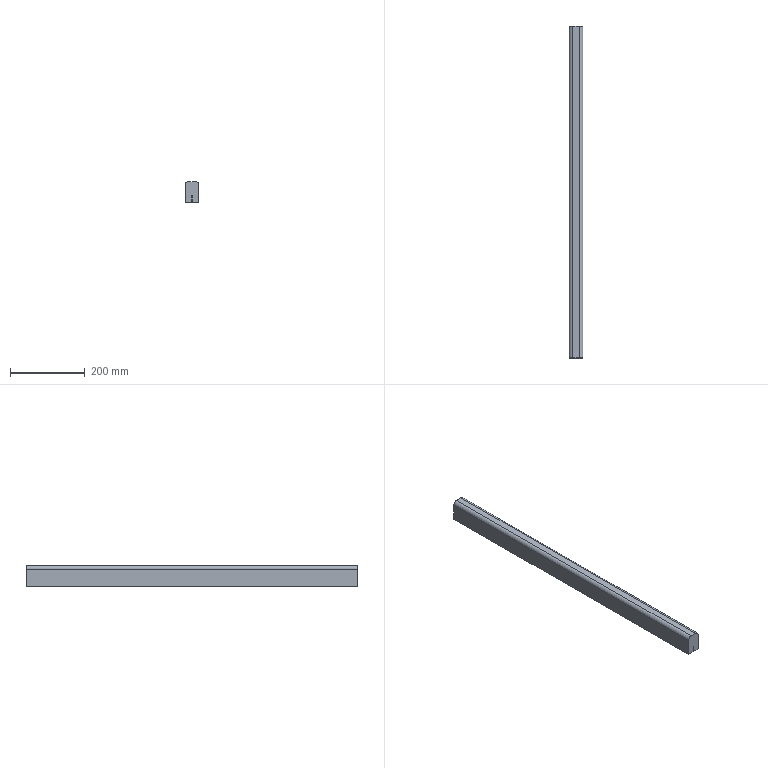Component | NX | CLOSING_ROD | 1 solid | 12 faces | box 37 x 889.3 x 56 mm | volume 1772451 mm3 | plane 10 | cylinder 2 | commonest cylinder face diameters 20 x2
STEP:
#1=CARTESIAN_POINT('',(0.,0.,0.));
#2=DIRECTION('',(0.,0.,1.));
#3=DIRECTION('',(1.,0.,0.));
#4=AXIS2_PLACEMENT_3D('',#1,#2,#3);
#5=CARTESIAN_POINT('',(344.,-444.651,-264.582));
#6=VERTEX_POINT('',#5);
#7=CARTESIAN_POINT('',(344.,444.651,-264.582));
#8=VERTEX_POINT('',#7);
#9=CARTESIAN_POINT('',(344.,-8359.443,-264.582));
#10=DIRECTION('',(0.,1.,0.));
#11=VECTOR('',#10,1.);
#12=LINE('',#9,#11);
#13=CARTESIAN_POINT('',(363.5,-8359.443,-264.582));
#14=DIRECTION('',(0.,0.,-1.));
#15=DIRECTION('',(-1.,0.,0.));
#16=AXIS2_PLACEMENT_3D('',#13,#14,#15);
#17=PLANE('',#16);
#18=CARTESIAN_POINT('',(19.5,0.));
#19=DIRECTION('',(0.,1.));
#20=VECTOR('',#19,1.);
#21=LINE('',#18,#20);
#22=(GEOMETRIC_REPRESENTATION_CONTEXT(2)PARAMETRIC_REPRESENTATION_CONTEXT()REPRESENTATION_CONTEXT('',''));
#23=DEFINITIONAL_REPRESENTATION('',(#21),#22);
#24=PCURVE('',#17,#23);
#25=CARTESIAN_POINT('',(344.,0.,-265.582));
#26=DIRECTION('',(-1.,0.,0.));
#27=DIRECTION('',(0.,0.,1.));
#28=AXIS2_PLACEMENT_3D('',#25,#26,#27);
#29=PLANE('',#28);
#30=CARTESIAN_POINT('',(1.,-8359.443));
#31=DIRECTION('',(0.,1.));
#32=VECTOR('',#31,1.);
#33=LINE('',#30,#32);
#34=(GEOMETRIC_REPRESENTATION_CONTEXT(2)PARAMETRIC_REPRESENTATION_CONTEXT()REPRESENTATION_CONTEXT('',''));
#35=DEFINITIONAL_REPRESENTATION('',(#33),#34);
#36=PCURVE('',#29,#35);
#37=SURFACE_CURVE('',#12,(#24,#36),.PCURVE_S1.);
#38=EDGE_CURVE('',#6,#8,#37,.T.);
#39=ORIENTED_EDGE('',*,*,#38,.F.);
#40=CARTESIAN_POINT('',(326.5,-444.651,-264.582));
#41=VERTEX_POINT('',#40);
#42=CARTESIAN_POINT('',(363.5,-444.651,-264.582));
#43=DIRECTION('',(1.,0.,0.));
#44=VECTOR('',#43,1.);
#45=LINE('',#42,#44);
#46=CARTESIAN_POINT('',(0.,7914.792));
#47=DIRECTION('',(-1.,0.));
#48=VECTOR('',#47,1.);
#49=LINE('',#46,#48);
#50=(GEOMETRIC_REPRESENTATION_CONTEXT(2)PARAMETRIC_REPRESENTATION_CONTEXT()REPRESENTATION_CONTEXT('',''));
#51=DEFINITIONAL_REPRESENTATION('',(#49),#50);
#52=PCURVE('',#17,#51);
#53=CARTESIAN_POINT('',(5.,-444.651,226.709));
#54=DIRECTION('',(0.,1.,0.));
#55=DIRECTION('',(0.,0.,1.));
#56=AXIS2_PLACEMENT_3D('',#53,#54,#55);
#57=PLANE('',#56);
#58=CARTESIAN_POINT('',(-491.291,358.5));
#59=DIRECTION('',(0.,1.));
#60=VECTOR('',#59,1.);
#61=LINE('',#58,#60);
#62=(GEOMETRIC_REPRESENTATION_CONTEXT(2)PARAMETRIC_REPRESENTATION_CONTEXT()REPRESENTATION_CONTEXT('',''));
#63=DEFINITIONAL_REPRESENTATION('',(#61),#62);
#64=PCURVE('',#57,#63);
#65=SURFACE_CURVE('',#45,(#52,#64),.PCURVE_S1.);
#66=EDGE_CURVE('',#41,#6,#65,.T.);
#67=ORIENTED_EDGE('',*,*,#66,.F.);
#68=CARTESIAN_POINT('',(326.5,444.651,-264.582));
#69=VERTEX_POINT('',#68);
#70=CARTESIAN_POINT('',(326.5,-8359.443,-264.582));
#71=DIRECTION('',(0.,1.,0.));
#72=VECTOR('',#71,1.);
#73=LINE('',#70,#72);
#74=CARTESIAN_POINT('',(37.,0.));
#75=DIRECTION('',(0.,1.));
#76=VECTOR('',#75,1.);
#77=LINE('',#74,#76);
#78=(GEOMETRIC_REPRESENTATION_CONTEXT(2)PARAMETRIC_REPRESENTATION_CONTEXT()REPRESENTATION_CONTEXT('',''));
#79=DEFINITIONAL_REPRESENTATION('',(#77),#78);
#80=PCURVE('',#17,#79);
#81=CARTESIAN_POINT('',(326.5,-8359.443,-249.582));
#82=DIRECTION('',(-1.,0.,0.));
#83=DIRECTION('',(0.,0.,1.));
#84=AXIS2_PLACEMENT_3D('',#81,#82,#83);
#85=PLANE('',#84);
#86=CARTESIAN_POINT('',(-15.,0.));
#87=DIRECTION('',(0.,1.));
#88=VECTOR('',#87,1.);
#89=LINE('',#86,#88);
#90=(GEOMETRIC_REPRESENTATION_CONTEXT(2)PARAMETRIC_REPRESENTATION_CONTEXT()REPRESENTATION_CONTEXT('',''));
#91=DEFINITIONAL_REPRESENTATION('',(#89),#90);
#92=PCURVE('',#85,#91);
#93=SURFACE_CURVE('',#73,(#80,#92),.PCURVE_S1.);
#94=EDGE_CURVE('',#41,#69,#93,.T.);
#95=ORIENTED_EDGE('',*,*,#94,.T.);
#96=CARTESIAN_POINT('',(363.5,444.651,-264.582));
#97=DIRECTION('',(-1.,0.,0.));
#98=VECTOR('',#97,1.);
#99=LINE('',#96,#98);
#100=CARTESIAN_POINT('',(0.,8804.095));
#101=DIRECTION('',(1.,0.));
#102=VECTOR('',#101,1.);
#103=LINE('',#100,#102);
#104=(GEOMETRIC_REPRESENTATION_CONTEXT(2)PARAMETRIC_REPRESENTATION_CONTEXT()REPRESENTATION_CONTEXT('',''));
#105=DEFINITIONAL_REPRESENTATION('',(#103),#104);
#106=PCURVE('',#17,#105);
#107=CARTESIAN_POINT('',(0.,444.651,0.));
#108=DIRECTION('',(0.,1.,0.));
#109=DIRECTION('',(0.,0.,1.));
#110=AXIS2_PLACEMENT_3D('',#107,#108,#109);
#111=PLANE('',#110);
#112=CARTESIAN_POINT('',(-264.582,363.5));
#113=DIRECTION('',(0.,-1.));
#114=VECTOR('',#113,1.);
#115=LINE('',#112,#114);
#116=(GEOMETRIC_REPRESENTATION_CONTEXT(2)PARAMETRIC_REPRESENTATION_CONTEXT()REPRESENTATION_CONTEXT('',''));
#117=DEFINITIONAL_REPRESENTATION('',(#115),#116);
#118=PCURVE('',#111,#117);
#119=SURFACE_CURVE('',#99,(#106,#118),.PCURVE_S1.);
#120=EDGE_CURVE('',#8,#69,#119,.T.);
#121=ORIENTED_EDGE('',*,*,#120,.F.);
#122=EDGE_LOOP('',(#39,#67,#95,#121));
#123=FACE_BOUND('',#122,.T.);
#124=ADVANCED_FACE('',(#123),#17,.T.);
#125=ORIENTED_EDGE('',*,*,#66,.T.);
#126=CARTESIAN_POINT('',(344.,-444.651,-246.582));
#127=VERTEX_POINT('',#126);
#128=CARTESIAN_POINT('',(344.,-444.651,226.709));
#129=DIRECTION('',(0.,0.,1.));
#130=VECTOR('',#129,1.);
#131=LINE('',#128,#130);
#132=CARTESIAN_POINT('',(0.,339.));
#133=DIRECTION('',(1.,0.));
#134=VECTOR('',#133,1.);
#135=LINE('',#132,#134);
#136=(GEOMETRIC_REPRESENTATION_CONTEXT(2)PARAMETRIC_REPRESENTATION_CONTEXT()REPRESENTATION_CONTEXT('',''));
#137=DEFINITIONAL_REPRESENTATION('',(#135),#136);
#138=PCURVE('',#57,#137);
#139=CARTESIAN_POINT('',(492.291,-444.651));
#140=DIRECTION('',(1.,0.));
#141=VECTOR('',#140,1.);
#142=LINE('',#139,#141);
#143=(GEOMETRIC_REPRESENTATION_CONTEXT(2)PARAMETRIC_REPRESENTATION_CONTEXT()REPRESENTATION_CONTEXT('',''));
#144=DEFINITIONAL_REPRESENTATION('',(#142),#143);
#145=PCURVE('',#29,#144);
#146=SURFACE_CURVE('',#131,(#138,#145),.PCURVE_S1.);
#147=EDGE_CURVE('',#6,#127,#146,.T.);
#148=ORIENTED_EDGE('',*,*,#147,.T.);
#149=CARTESIAN_POINT('',(346.,-444.651,-246.582));
#150=VERTEX_POINT('',#149);
#151=CARTESIAN_POINT('',(5.,-444.651,-246.582));
#152=DIRECTION('',(1.,0.,0.));
#153=VECTOR('',#152,1.);
#154=LINE('',#151,#153);
#155=CARTESIAN_POINT('',(-473.291,0.));
#156=DIRECTION('',(0.,1.));
#157=VECTOR('',#156,1.);
#158=LINE('',#155,#157);
#159=(GEOMETRIC_REPRESENTATION_CONTEXT(2)PARAMETRIC_REPRESENTATION_CONTEXT()REPRESENTATION_CONTEXT('',''));
#160=DEFINITIONAL_REPRESENTATION('',(#158),#159);
#161=PCURVE('',#57,#160);
#162=CARTESIAN_POINT('',(345.,0.,-246.582));
#163=DIRECTION('',(0.,0.,1.));
#164=DIRECTION('',(1.,0.,0.));
#165=AXIS2_PLACEMENT_3D('',#162,#163,#164);
#166=PLANE('',#165);
#167=CARTESIAN_POINT('',(-340.,-444.651));
#168=DIRECTION('',(1.,0.));
#169=VECTOR('',#168,1.);
#170=LINE('',#167,#169);
#171=(GEOMETRIC_REPRESENTATION_CONTEXT(2)PARAMETRIC_REPRESENTATION_CONTEXT()REPRESENTATION_CONTEXT('',''));
#172=DEFINITIONAL_REPRESENTATION('',(#170),#171);
#173=PCURVE('',#166,#172);
#174=SURFACE_CURVE('',#154,(#161,#173),.PCURVE_S1.);
#175=EDGE_CURVE('',#127,#150,#174,.T.);
#176=ORIENTED_EDGE('',*,*,#175,.T.);
#177=CARTESIAN_POINT('',(346.,-444.651,-264.582));
#178=VERTEX_POINT('',#177);
#179=CARTESIAN_POINT('',(346.,-444.651,226.709));
#180=DIRECTION('',(0.,0.,-1.));
#181=VECTOR('',#180,1.);
#182=LINE('',#179,#181);
#183=CARTESIAN_POINT('',(0.,341.));
#184=DIRECTION('',(-1.,0.));
#185=VECTOR('',#184,1.);
#186=LINE('',#183,#185);
#187=(GEOMETRIC_REPRESENTATION_CONTEXT(2)PARAMETRIC_REPRESENTATION_CONTEXT()REPRESENTATION_CONTEXT('',''));
#188=DEFINITIONAL_REPRESENTATION('',(#186),#187);
#189=PCURVE('',#57,#188);
#190=CARTESIAN_POINT('',(346.,0.,-265.582));
#191=DIRECTION('',(1.,0.,0.));
#192=DIRECTION('',(0.,0.,-1.));
#193=AXIS2_PLACEMENT_3D('',#190,#191,#192);
#194=PLANE('',#193);
#195=CARTESIAN_POINT('',(-492.291,-444.651));
#196=DIRECTION('',(1.,0.));
#197=VECTOR('',#196,1.);
#198=LINE('',#195,#197);
#199=(GEOMETRIC_REPRESENTATION_CONTEXT(2)PARAMETRIC_REPRESENTATION_CONTEXT()REPRESENTATION_CONTEXT('',''));
#200=DEFINITIONAL_REPRESENTATION('',(#198),#199);
#201=PCURVE('',#194,#200);
#202=SURFACE_CURVE('',#182,(#189,#201),.PCURVE_S1.);
#203=EDGE_CURVE('',#150,#178,#202,.T.);
#204=ORIENTED_EDGE('',*,*,#203,.T.);
#205=CARTESIAN_POINT('',(363.5,-444.651,-264.582));
#206=VERTEX_POINT('',#205);
#207=CARTESIAN_POINT('',(363.5,-444.651,-264.582));
#208=DIRECTION('',(1.,0.,0.));
#209=VECTOR('',#208,1.);
#210=LINE('',#207,#209);
#211=CARTESIAN_POINT('',(-491.291,358.5));
#212=DIRECTION('',(0.,1.));
#213=VECTOR('',#212,1.);
#214=LINE('',#211,#213);
#215=(GEOMETRIC_REPRESENTATION_CONTEXT(2)PARAMETRIC_REPRESENTATION_CONTEXT()REPRESENTATION_CONTEXT('',''));
#216=DEFINITIONAL_REPRESENTATION('',(#214),#215);
#217=PCURVE('',#57,#216);
#218=CARTESIAN_POINT('',(363.5,-8359.443,-264.582));
#219=DIRECTION('',(0.,0.,-1.));
#220=DIRECTION('',(-1.,0.,0.));
#221=AXIS2_PLACEMENT_3D('',#218,#219,#220);
#222=PLANE('',#221);
#223=CARTESIAN_POINT('',(0.,7914.792));
#224=DIRECTION('',(-1.,0.));
#225=VECTOR('',#224,1.);
#226=LINE('',#223,#225);
#227=(GEOMETRIC_REPRESENTATION_CONTEXT(2)PARAMETRIC_REPRESENTATION_CONTEXT()REPRESENTATION_CONTEXT('',''));
#228=DEFINITIONAL_REPRESENTATION('',(#226),#227);
#229=PCURVE('',#222,#228);
#230=SURFACE_CURVE('',#210,(#217,#229),.PCURVE_S1.);
#231=EDGE_CURVE('',#178,#206,#230,.T.);
#232=ORIENTED_EDGE('',*,*,#231,.T.);
#233=CARTESIAN_POINT('',(363.5,-444.651,-218.582));
#234=VERTEX_POINT('',#233);
#235=CARTESIAN_POINT('',(363.5,-444.651,-208.582));
#236=DIRECTION('',(0.,0.,1.));
#237=VECTOR('',#236,1.);
#238=LINE('',#235,#237);
#239=CARTESIAN_POINT('',(-435.291,358.5));
#240=DIRECTION('',(1.,0.));
#241=VECTOR('',#240,1.);
#242=LINE('',#239,#241);
#243=(GEOMETRIC_REPRESENTATION_CONTEXT(2)PARAMETRIC_REPRESENTATION_CONTEXT()REPRESENTATION_CONTEXT('',''));
#244=DEFINITIONAL_REPRESENTATION('',(#242),#243);
#245=PCURVE('',#57,#244);
#246=CARTESIAN_POINT('',(363.5,-8359.443,-208.582));
#247=DIRECTION('',(1.,0.,0.));
#248=DIRECTION('',(0.,0.,-1.));
#249=AXIS2_PLACEMENT_3D('',#246,#247,#248);
#250=PLANE('',#249);
#251=CARTESIAN_POINT('',(0.,7914.792));
#252=DIRECTION('',(-1.,0.));
#253=VECTOR('',#252,1.);
#254=LINE('',#251,#253);
#255=(GEOMETRIC_REPRESENTATION_CONTEXT(2)PARAMETRIC_REPRESENTATION_CONTEXT()REPRESENTATION_CONTEXT('',''));
#256=DEFINITIONAL_REPRESENTATION('',(#254),#255);
#257=PCURVE('',#250,#256);
#258=SURFACE_CURVE('',#238,(#245,#257),.PCURVE_S1.);
#259=EDGE_CURVE('',#206,#234,#258,.T.);
#260=ORIENTED_EDGE('',*,*,#259,.T.);
#261=CARTESIAN_POINT('',(353.5,-444.651,-208.582));
#262=VERTEX_POINT('',#261);
#263=CARTESIAN_POINT('',(353.5,-444.651,-218.582));
#264=DIRECTION('',(0.,-1.,0.));
#265=DIRECTION('',(0.,0.,1.));
#266=AXIS2_PLACEMENT_3D('',#263,#264,#265);
#267=CIRCLE('',#266,10.);
#268=CARTESIAN_POINT('',(-435.291,348.5));
#269=CARTESIAN_POINT('',(-435.291,331.179));
#270=CARTESIAN_POINT('',(-450.291,339.84));
#271=CARTESIAN_POINT('',(-465.291,348.5));
#272=CARTESIAN_POINT('',(-450.291,357.16));
#273=CARTESIAN_POINT('',(-435.291,365.821));
#274=CARTESIAN_POINT('',(-435.291,348.5));
#275=(BOUNDED_CURVE()B_SPLINE_CURVE(2,(#268,#269,#270,#271,#272,#273,#274),.UNSPECIFIED.,.T.,.F.)B_SPLINE_CURVE_WITH_KNOTS((1,2,2,2,2,1),(-2.094,0.,2.094,4.189,6.283,8.378),.UNSPECIFIED.)CURVE()GEOMETRIC_REPRESENTATION_ITEM()RATIONAL_B_SPLINE_CURVE((1.,0.5,1.,0.5,1.,0.5,1.))REPRESENTATION_ITEM(''));
#276=(GEOMETRIC_REPRESENTATION_CONTEXT(2)PARAMETRIC_REPRESENTATION_CONTEXT()REPRESENTATION_CONTEXT('',''));
#277=DEFINITIONAL_REPRESENTATION('',(#275),#276);
#278=PCURVE('',#57,#277);
#279=CARTESIAN_POINT('',(353.5,-8359.443,-218.582));
#280=DIRECTION('',(0.,1.,0.));
#281=DIRECTION('',(0.,0.,1.));
#282=AXIS2_PLACEMENT_3D('',#279,#280,#281);
#283=CYLINDRICAL_SURFACE('',#282,10.);
#284=CARTESIAN_POINT('',(6.283,7914.792));
#285=DIRECTION('',(-1.,0.));
#286=VECTOR('',#285,1.);
#287=LINE('',#284,#286);
#288=(GEOMETRIC_REPRESENTATION_CONTEXT(2)PARAMETRIC_REPRESENTATION_CONTEXT()REPRESENTATION_CONTEXT('',''));
#289=DEFINITIONAL_REPRESENTATION('',(#287),#288);
#290=PCURVE('',#283,#289);
#291=SURFACE_CURVE('',#267,(#278,#290),.PCURVE_S1.);
#292=EDGE_CURVE('',#234,#262,#291,.T.);
#293=ORIENTED_EDGE('',*,*,#292,.T.);
#294=CARTESIAN_POINT('',(336.5,-444.651,-208.582));
#295=VERTEX_POINT('',#294);
#296=CARTESIAN_POINT('',(326.5,-444.651,-208.582));
#297=DIRECTION('',(-1.,0.,0.));
#298=VECTOR('',#297,1.);
#299=LINE('',#296,#298);
#300=CARTESIAN_POINT('',(-435.291,321.5));
#301=DIRECTION('',(0.,-1.));
#302=VECTOR('',#301,1.);
#303=LINE('',#300,#302);
#304=(GEOMETRIC_REPRESENTATION_CONTEXT(2)PARAMETRIC_REPRESENTATION_CONTEXT()REPRESENTATION_CONTEXT('',''));
#305=DEFINITIONAL_REPRESENTATION('',(#303),#304);
#306=PCURVE('',#57,#305);
#307=CARTESIAN_POINT('',(326.5,-8359.443,-208.582));
#308=DIRECTION('',(0.,0.,1.));
#309=DIRECTION('',(1.,0.,0.));
#310=AXIS2_PLACEMENT_3D('',#307,#308,#309);
#311=PLANE('',#310);
#312=CARTESIAN_POINT('',(0.,7914.792));
#313=DIRECTION('',(-1.,0.));
#314=VECTOR('',#313,1.);
#315=LINE('',#312,#314);
#316=(GEOMETRIC_REPRESENTATION_CONTEXT(2)PARAMETRIC_REPRESENTATION_CONTEXT()REPRESENTATION_CONTEXT('',''));
#317=DEFINITIONAL_REPRESENTATION('',(#315),#316);
#318=PCURVE('',#311,#317);
#319=SURFACE_CURVE('',#299,(#306,#318),.PCURVE_S1.);
#320=EDGE_CURVE('',#262,#295,#319,.T.);
#321=ORIENTED_EDGE('',*,*,#320,.T.);
#322=CARTESIAN_POINT('',(326.5,-444.651,-218.582));
#323=VERTEX_POINT('',#322);
#324=CARTESIAN_POINT('',(336.5,-444.651,-218.582));
#325=DIRECTION('',(0.,-1.,0.));
#326=DIRECTION('',(0.,0.,1.));
#327=AXIS2_PLACEMENT_3D('',#324,#325,#326);
#328=CIRCLE('',#327,10.);
#329=CARTESIAN_POINT('',(-435.291,331.5));
#330=CARTESIAN_POINT('',(-435.291,314.179));
#331=CARTESIAN_POINT('',(-450.291,322.84));
#332=CARTESIAN_POINT('',(-465.291,331.5));
#333=CARTESIAN_POINT('',(-450.291,340.16));
#334=CARTESIAN_POINT('',(-435.291,348.821));
#335=CARTESIAN_POINT('',(-435.291,331.5));
#336=(BOUNDED_CURVE()B_SPLINE_CURVE(2,(#329,#330,#331,#332,#333,#334,#335),.UNSPECIFIED.,.T.,.F.)B_SPLINE_CURVE_WITH_KNOTS((1,2,2,2,2,1),(-2.094,0.,2.094,4.189,6.283,8.378),.UNSPECIFIED.)CURVE()GEOMETRIC_REPRESENTATION_ITEM()RATIONAL_B_SPLINE_CURVE((1.,0.5,1.,0.5,1.,0.5,1.))REPRESENTATION_ITEM(''));
#337=(GEOMETRIC_REPRESENTATION_CONTEXT(2)PARAMETRIC_REPRESENTATION_CONTEXT()REPRESENTATION_CONTEXT('',''));
#338=DEFINITIONAL_REPRESENTATION('',(#336),#337);
#339=PCURVE('',#57,#338);
#340=CARTESIAN_POINT('',(336.5,-8359.443,-218.582));
#341=DIRECTION('',(0.,1.,0.));
#342=DIRECTION('',(0.,0.,1.));
#343=AXIS2_PLACEMENT_3D('',#340,#341,#342);
#344=CYLINDRICAL_SURFACE('',#343,10.);
#345=CARTESIAN_POINT('',(6.283,7914.792));
#346=DIRECTION('',(-1.,0.));
#347=VECTOR('',#346,1.);
#348=LINE('',#345,#347);
#349=(GEOMETRIC_REPRESENTATION_CONTEXT(2)PARAMETRIC_REPRESENTATION_CONTEXT()REPRESENTATION_CONTEXT('',''));
#350=DEFINITIONAL_REPRESENTATION('',(#348),#349);
#351=PCURVE('',#344,#350);
#352=SURFACE_CURVE('',#328,(#339,#351),.PCURVE_S1.);
#353=EDGE_CURVE('',#295,#323,#352,.T.);
#354=ORIENTED_EDGE('',*,*,#353,.T.);
#355=CARTESIAN_POINT('',(326.5,-444.651,-249.582));
#356=DIRECTION('',(0.,0.,-1.));
#357=VECTOR('',#356,1.);
#358=LINE('',#355,#357);
#359=CARTESIAN_POINT('',(-476.291,321.5));
#360=DIRECTION('',(-1.,0.));
#361=VECTOR('',#360,1.);
#362=LINE('',#359,#361);
#363=(GEOMETRIC_REPRESENTATION_CONTEXT(2)PARAMETRIC_REPRESENTATION_CONTEXT()REPRESENTATION_CONTEXT('',''));
#364=DEFINITIONAL_REPRESENTATION('',(#362),#363);
#365=PCURVE('',#57,#364);
#366=CARTESIAN_POINT('',(0.,7914.792));
#367=DIRECTION('',(-1.,0.));
#368=VECTOR('',#367,1.);
#369=LINE('',#366,#368);
#370=(GEOMETRIC_REPRESENTATION_CONTEXT(2)PARAMETRIC_REPRESENTATION_CONTEXT()REPRESENTATION_CONTEXT('',''));
#371=DEFINITIONAL_REPRESENTATION('',(#369),#370);
#372=PCURVE('',#85,#371);
#373=SURFACE_CURVE('',#358,(#365,#372),.PCURVE_S1.);
#374=EDGE_CURVE('',#323,#41,#373,.T.);
#375=ORIENTED_EDGE('',*,*,#374,.T.);
#376=EDGE_LOOP('',(#125,#148,#176,#204,#232,#260,#293,#321,#354,#375));
#377=FACE_BOUND('',#376,.T.);
#378=ADVANCED_FACE('',(#377),#57,.F.);
#379=CARTESIAN_POINT('',(336.5,444.651,-208.582));
#380=VERTEX_POINT('',#379);
#381=CARTESIAN_POINT('',(353.5,444.651,-208.582));
#382=VERTEX_POINT('',#381);
#383=CARTESIAN_POINT('',(326.5,444.651,-208.582));
#384=DIRECTION('',(1.,0.,0.));
#385=VECTOR('',#384,1.);
#386=LINE('',#383,#385);
#387=CARTESIAN_POINT('',(0.,8804.095));
#388=DIRECTION('',(1.,0.));
#389=VECTOR('',#388,1.);
#390=LINE('',#387,#389);
#391=(GEOMETRIC_REPRESENTATION_CONTEXT(2)PARAMETRIC_REPRESENTATION_CONTEXT()REPRESENTATION_CONTEXT('',''));
#392=DEFINITIONAL_REPRESENTATION('',(#390),#391);
#393=PCURVE('',#311,#392);
#394=CARTESIAN_POINT('',(-208.582,326.5));
#395=DIRECTION('',(0.,1.));
#396=VECTOR('',#395,1.);
#397=LINE('',#394,#396);
#398=(GEOMETRIC_REPRESENTATION_CONTEXT(2)PARAMETRIC_REPRESENTATION_CONTEXT()REPRESENTATION_CONTEXT('',''));
#399=DEFINITIONAL_REPRESENTATION('',(#397),#398);
#400=PCURVE('',#111,#399);
#401=SURFACE_CURVE('',#386,(#393,#400),.PCURVE_S1.);
#402=EDGE_CURVE('',#380,#382,#401,.T.);
#403=ORIENTED_EDGE('',*,*,#402,.F.);
#404=CARTESIAN_POINT('',(336.5,-8359.443,-208.582));
#405=DIRECTION('',(0.,-1.,0.));
#406=VECTOR('',#405,1.);
#407=LINE('',#404,#406);
#408=CARTESIAN_POINT('',(10.,0.));
#409=DIRECTION('',(0.,-1.));
#410=VECTOR('',#409,1.);
#411=LINE('',#408,#410);
#412=(GEOMETRIC_REPRESENTATION_CONTEXT(2)PARAMETRIC_REPRESENTATION_CONTEXT()REPRESENTATION_CONTEXT('',''));
#413=DEFINITIONAL_REPRESENTATION('',(#411),#412);
#414=PCURVE('',#311,#413);
#415=CARTESIAN_POINT('',(6.283,0.));
#416=DIRECTION('',(0.,-1.));
#417=VECTOR('',#416,1.);
#418=LINE('',#415,#417);
#419=(GEOMETRIC_REPRESENTATION_CONTEXT(2)PARAMETRIC_REPRESENTATION_CONTEXT()REPRESENTATION_CONTEXT('',''));
#420=DEFINITIONAL_REPRESENTATION('',(#418),#419);
#421=PCURVE('',#344,#420);
#422=SURFACE_CURVE('',#407,(#414,#421),.PCURVE_S1.);
#423=EDGE_CURVE('',#380,#295,#422,.T.);
#424=ORIENTED_EDGE('',*,*,#423,.T.);
#425=ORIENTED_EDGE('',*,*,#320,.F.);
#426=CARTESIAN_POINT('',(353.5,-8359.443,-208.582));
#427=DIRECTION('',(0.,1.,0.));
#428=VECTOR('',#427,1.);
#429=LINE('',#426,#428);
#430=CARTESIAN_POINT('',(27.,0.));
#431=DIRECTION('',(0.,1.));
#432=VECTOR('',#431,1.);
#433=LINE('',#430,#432);
#434=(GEOMETRIC_REPRESENTATION_CONTEXT(2)PARAMETRIC_REPRESENTATION_CONTEXT()REPRESENTATION_CONTEXT('',''));
#435=DEFINITIONAL_REPRESENTATION('',(#433),#434);
#436=PCURVE('',#311,#435);
#437=CARTESIAN_POINT('',(0.,0.));
#438=DIRECTION('',(0.,1.));
#439=VECTOR('',#438,1.);
#440=LINE('',#437,#439);
#441=(GEOMETRIC_REPRESENTATION_CONTEXT(2)PARAMETRIC_REPRESENTATION_CONTEXT()REPRESENTATION_CONTEXT('',''));
#442=DEFINITIONAL_REPRESENTATION('',(#440),#441);
#443=PCURVE('',#283,#442);
#444=SURFACE_CURVE('',#429,(#436,#443),.PCURVE_S1.);
#445=EDGE_CURVE('',#262,#382,#444,.T.);
#446=ORIENTED_EDGE('',*,*,#445,.T.);
#447=EDGE_LOOP('',(#403,#424,#425,#446));
#448=FACE_BOUND('',#447,.T.);
#449=ADVANCED_FACE('',(#448),#311,.T.);
#450=CARTESIAN_POINT('',(363.5,444.651,-218.582));
#451=VERTEX_POINT('',#450);
#452=CARTESIAN_POINT('',(363.5,444.651,-264.582));
#453=VERTEX_POINT('',#452);
#454=CARTESIAN_POINT('',(363.5,444.651,-208.582));
#455=DIRECTION('',(0.,0.,-1.));
#456=VECTOR('',#455,1.);
#457=LINE('',#454,#456);
#458=CARTESIAN_POINT('',(0.,8804.095));
#459=DIRECTION('',(1.,0.));
#460=VECTOR('',#459,1.);
#461=LINE('',#458,#460);
#462=(GEOMETRIC_REPRESENTATION_CONTEXT(2)PARAMETRIC_REPRESENTATION_CONTEXT()REPRESENTATION_CONTEXT('',''));
#463=DEFINITIONAL_REPRESENTATION('',(#461),#462);
#464=PCURVE('',#250,#463);
#465=CARTESIAN_POINT('',(-208.582,363.5));
#466=DIRECTION('',(-1.,0.));
#467=VECTOR('',#466,1.);
#468=LINE('',#465,#467);
#469=(GEOMETRIC_REPRESENTATION_CONTEXT(2)PARAMETRIC_REPRESENTATION_CONTEXT()REPRESENTATION_CONTEXT('',''));
#470=DEFINITIONAL_REPRESENTATION('',(#468),#469);
#471=PCURVE('',#111,#470);
#472=SURFACE_CURVE('',#457,(#464,#471),.PCURVE_S1.);
#473=EDGE_CURVE('',#451,#453,#472,.T.);
#474=ORIENTED_EDGE('',*,*,#473,.F.);
#475=CARTESIAN_POINT('',(363.5,-8359.443,-218.582));
#476=DIRECTION('',(0.,-1.,0.));
#477=VECTOR('',#476,1.);
#478=LINE('',#475,#477);
#479=CARTESIAN_POINT('',(10.,0.));
#480=DIRECTION('',(0.,-1.));
#481=VECTOR('',#480,1.);
#482=LINE('',#479,#481);
#483=(GEOMETRIC_REPRESENTATION_CONTEXT(2)PARAMETRIC_REPRESENTATION_CONTEXT()REPRESENTATION_CONTEXT('',''));
#484=DEFINITIONAL_REPRESENTATION('',(#482),#483);
#485=PCURVE('',#250,#484);
#486=CARTESIAN_POINT('',(1.571,0.));
#487=DIRECTION('',(0.,-1.));
#488=VECTOR('',#487,1.);
#489=LINE('',#486,#488);
#490=(GEOMETRIC_REPRESENTATION_CONTEXT(2)PARAMETRIC_REPRESENTATION_CONTEXT()REPRESENTATION_CONTEXT('',''));
#491=DEFINITIONAL_REPRESENTATION('',(#489),#490);
#492=PCURVE('',#283,#491);
#493=SURFACE_CURVE('',#478,(#485,#492),.PCURVE_S1.);
#494=EDGE_CURVE('',#451,#234,#493,.T.);
#495=ORIENTED_EDGE('',*,*,#494,.T.);
#496=ORIENTED_EDGE('',*,*,#259,.F.);
#497=CARTESIAN_POINT('',(363.5,-8359.443,-264.582));
#498=DIRECTION('',(0.,1.,0.));
#499=VECTOR('',#498,1.);
#500=LINE('',#497,#499);
#501=CARTESIAN_POINT('',(56.,0.));
#502=DIRECTION('',(0.,1.));
#503=VECTOR('',#502,1.);
#504=LINE('',#501,#503);
#505=(GEOMETRIC_REPRESENTATION_CONTEXT(2)PARAMETRIC_REPRESENTATION_CONTEXT()REPRESENTATION_CONTEXT('',''));
#506=DEFINITIONAL_REPRESENTATION('',(#504),#505);
#507=PCURVE('',#250,#506);
#508=CARTESIAN_POINT('',(0.,0.));
#509=DIRECTION('',(0.,1.));
#510=VECTOR('',#509,1.);
#511=LINE('',#508,#510);
#512=(GEOMETRIC_REPRESENTATION_CONTEXT(2)PARAMETRIC_REPRESENTATION_CONTEXT()REPRESENTATION_CONTEXT('',''));
#513=DEFINITIONAL_REPRESENTATION('',(#511),#512);
#514=PCURVE('',#222,#513);
#515=SURFACE_CURVE('',#500,(#507,#514),.PCURVE_S1.);
#516=EDGE_CURVE('',#206,#453,#515,.T.);
#517=ORIENTED_EDGE('',*,*,#516,.T.);
#518=EDGE_LOOP('',(#474,#495,#496,#517));
#519=FACE_BOUND('',#518,.T.);
#520=ADVANCED_FACE('',(#519),#250,.T.);
#521=CARTESIAN_POINT('',(346.,444.651,-264.582));
#522=VERTEX_POINT('',#521);
#523=CARTESIAN_POINT('',(346.,-8359.443,-264.582));
#524=DIRECTION('',(0.,-1.,0.));
#525=VECTOR('',#524,1.);
#526=LINE('',#523,#525);
#527=CARTESIAN_POINT('',(17.5,0.));
#528=DIRECTION('',(0.,-1.));
#529=VECTOR('',#528,1.);
#530=LINE('',#527,#529);
#531=(GEOMETRIC_REPRESENTATION_CONTEXT(2)PARAMETRIC_REPRESENTATION_CONTEXT()REPRESENTATION_CONTEXT('',''));
#532=DEFINITIONAL_REPRESENTATION('',(#530),#531);
#533=PCURVE('',#222,#532);
#534=CARTESIAN_POINT('',(-1.,-8359.443));
#535=DIRECTION('',(0.,-1.));
#536=VECTOR('',#535,1.);
#537=LINE('',#534,#536);
#538=(GEOMETRIC_REPRESENTATION_CONTEXT(2)PARAMETRIC_REPRESENTATION_CONTEXT()REPRESENTATION_CONTEXT('',''));
#539=DEFINITIONAL_REPRESENTATION('',(#537),#538);
#540=PCURVE('',#194,#539);
#541=SURFACE_CURVE('',#526,(#533,#540),.PCURVE_S1.);
#542=EDGE_CURVE('',#522,#178,#541,.T.);
#543=ORIENTED_EDGE('',*,*,#542,.F.);
#544=CARTESIAN_POINT('',(363.5,444.651,-264.582));
#545=DIRECTION('',(-1.,0.,0.));
#546=VECTOR('',#545,1.);
#547=LINE('',#544,#546);
#548=CARTESIAN_POINT('',(0.,8804.095));
#549=DIRECTION('',(1.,0.));
#550=VECTOR('',#549,1.);
#551=LINE('',#548,#550);
#552=(GEOMETRIC_REPRESENTATION_CONTEXT(2)PARAMETRIC_REPRESENTATION_CONTEXT()REPRESENTATION_CONTEXT('',''));
#553=DEFINITIONAL_REPRESENTATION('',(#551),#552);
#554=PCURVE('',#222,#553);
#555=CARTESIAN_POINT('',(-264.582,363.5));
#556=DIRECTION('',(0.,-1.));
#557=VECTOR('',#556,1.);
#558=LINE('',#555,#557);
#559=(GEOMETRIC_REPRESENTATION_CONTEXT(2)PARAMETRIC_REPRESENTATION_CONTEXT()REPRESENTATION_CONTEXT('',''));
#560=DEFINITIONAL_REPRESENTATION('',(#558),#559);
#561=PCURVE('',#111,#560);
#562=SURFACE_CURVE('',#547,(#554,#561),.PCURVE_S1.);
#563=EDGE_CURVE('',#453,#522,#562,.T.);
#564=ORIENTED_EDGE('',*,*,#563,.F.);
#565=ORIENTED_EDGE('',*,*,#516,.F.);
#566=ORIENTED_EDGE('',*,*,#231,.F.);
#567=EDGE_LOOP('',(#543,#564,#565,#566));
#568=FACE_BOUND('',#567,.T.);
#569=ADVANCED_FACE('',(#568),#222,.T.);
#570=ORIENTED_EDGE('',*,*,#374,.F.);
#571=CARTESIAN_POINT('',(326.5,444.651,-218.582));
#572=VERTEX_POINT('',#571);
#573=CARTESIAN_POINT('',(326.5,-8359.443,-218.582));
#574=DIRECTION('',(0.,1.,0.));
#575=VECTOR('',#574,1.);
#576=LINE('',#573,#575);
#577=CARTESIAN_POINT('',(31.,0.));
#578=DIRECTION('',(0.,1.));
#579=VECTOR('',#578,1.);
#580=LINE('',#577,#579);
#581=(GEOMETRIC_REPRESENTATION_CONTEXT(2)PARAMETRIC_REPRESENTATION_CONTEXT()REPRESENTATION_CONTEXT('',''));
#582=DEFINITIONAL_REPRESENTATION('',(#580),#581);
#583=PCURVE('',#85,#582);
#584=CARTESIAN_POINT('',(4.712,0.));
#585=DIRECTION('',(0.,1.));
#586=VECTOR('',#585,1.);
#587=LINE('',#584,#586);
#588=(GEOMETRIC_REPRESENTATION_CONTEXT(2)PARAMETRIC_REPRESENTATION_CONTEXT()REPRESENTATION_CONTEXT('',''));
#589=DEFINITIONAL_REPRESENTATION('',(#587),#588);
#590=PCURVE('',#344,#589);
#591=SURFACE_CURVE('',#576,(#583,#590),.PCURVE_S1.);
#592=EDGE_CURVE('',#323,#572,#591,.T.);
#593=ORIENTED_EDGE('',*,*,#592,.T.);
#594=CARTESIAN_POINT('',(326.5,444.651,-249.582));
#595=DIRECTION('',(0.,0.,1.));
#596=VECTOR('',#595,1.);
#597=LINE('',#594,#596);
#598=CARTESIAN_POINT('',(0.,8804.095));
#599=DIRECTION('',(1.,0.));
#600=VECTOR('',#599,1.);
#601=LINE('',#598,#600);
#602=(GEOMETRIC_REPRESENTATION_CONTEXT(2)PARAMETRIC_REPRESENTATION_CONTEXT()REPRESENTATION_CONTEXT('',''));
#603=DEFINITIONAL_REPRESENTATION('',(#601),#602);
#604=PCURVE('',#85,#603);
#605=CARTESIAN_POINT('',(-249.582,326.5));
#606=DIRECTION('',(1.,0.));
#607=VECTOR('',#606,1.);
#608=LINE('',#605,#607);
#609=(GEOMETRIC_REPRESENTATION_CONTEXT(2)PARAMETRIC_REPRESENTATION_CONTEXT()REPRESENTATION_CONTEXT('',''));
#610=DEFINITIONAL_REPRESENTATION('',(#608),#609);
#611=PCURVE('',#111,#610);
#612=SURFACE_CURVE('',#597,(#604,#611),.PCURVE_S1.);
#613=EDGE_CURVE('',#69,#572,#612,.T.);
#614=ORIENTED_EDGE('',*,*,#613,.F.);
#615=ORIENTED_EDGE('',*,*,#94,.F.);
#616=EDGE_LOOP('',(#570,#593,#614,#615));
#617=FACE_BOUND('',#616,.T.);
#618=ADVANCED_FACE('',(#617),#85,.T.);
#619=CARTESIAN_POINT('',(344.,444.651,-246.582));
#620=VERTEX_POINT('',#619);
#621=CARTESIAN_POINT('',(344.,444.651,0.));
#622=DIRECTION('',(0.,0.,1.));
#623=VECTOR('',#622,1.);
#624=LINE('',#621,#623);
#625=CARTESIAN_POINT('',(0.,344.));
#626=DIRECTION('',(1.,0.));
#627=VECTOR('',#626,1.);
#628=LINE('',#625,#627);
#629=(GEOMETRIC_REPRESENTATION_CONTEXT(2)PARAMETRIC_REPRESENTATION_CONTEXT()REPRESENTATION_CONTEXT('',''));
#630=DEFINITIONAL_REPRESENTATION('',(#628),#629);
#631=PCURVE('',#111,#630);
#632=CARTESIAN_POINT('',(265.582,444.651));
#633=DIRECTION('',(1.,0.));
#634=VECTOR('',#633,1.);
#635=LINE('',#632,#634);
#636=(GEOMETRIC_REPRESENTATION_CONTEXT(2)PARAMETRIC_REPRESENTATION_CONTEXT()REPRESENTATION_CONTEXT('',''));
#637=DEFINITIONAL_REPRESENTATION('',(#635),#636);
#638=PCURVE('',#29,#637);
#639=SURFACE_CURVE('',#624,(#631,#638),.PCURVE_S1.);
#640=EDGE_CURVE('',#8,#620,#639,.T.);
#641=ORIENTED_EDGE('',*,*,#640,.F.);
#642=ORIENTED_EDGE('',*,*,#120,.T.);
#643=ORIENTED_EDGE('',*,*,#613,.T.);
#644=CARTESIAN_POINT('',(336.5,444.651,-218.582));
#645=DIRECTION('',(0.,1.,0.));
#646=DIRECTION('',(0.,0.,1.));
#647=AXIS2_PLACEMENT_3D('',#644,#645,#646);
#648=CIRCLE('',#647,10.);
#649=CARTESIAN_POINT('',(-218.582,336.5));
#650=DIRECTION('',(1.,0.));
#651=AXIS2_PLACEMENT_2D('',#649,#650);
#652=CIRCLE('',#651,10.);
#653=(GEOMETRIC_REPRESENTATION_CONTEXT(2)PARAMETRIC_REPRESENTATION_CONTEXT()REPRESENTATION_CONTEXT('',''));
#654=DEFINITIONAL_REPRESENTATION('',(#652),#653);
#655=PCURVE('',#111,#654);
#656=CARTESIAN_POINT('',(0.,8804.095));
#657=DIRECTION('',(1.,0.));
#658=VECTOR('',#657,1.);
#659=LINE('',#656,#658);
#660=(GEOMETRIC_REPRESENTATION_CONTEXT(2)PARAMETRIC_REPRESENTATION_CONTEXT()REPRESENTATION_CONTEXT('',''));
#661=DEFINITIONAL_REPRESENTATION('',(#659),#660);
#662=PCURVE('',#344,#661);
#663=SURFACE_CURVE('',#648,(#655,#662),.PCURVE_S1.);
#664=EDGE_CURVE('',#572,#380,#663,.T.);
#665=ORIENTED_EDGE('',*,*,#664,.T.);
#666=ORIENTED_EDGE('',*,*,#402,.T.);
#667=CARTESIAN_POINT('',(353.5,444.651,-218.582));
#668=DIRECTION('',(0.,1.,0.));
#669=DIRECTION('',(0.,0.,1.));
#670=AXIS2_PLACEMENT_3D('',#667,#668,#669);
#671=CIRCLE('',#670,10.);
#672=CARTESIAN_POINT('',(-218.582,353.5));
#673=DIRECTION('',(1.,0.));
#674=AXIS2_PLACEMENT_2D('',#672,#673);
#675=CIRCLE('',#674,10.);
#676=(GEOMETRIC_REPRESENTATION_CONTEXT(2)PARAMETRIC_REPRESENTATION_CONTEXT()REPRESENTATION_CONTEXT('',''));
#677=DEFINITIONAL_REPRESENTATION('',(#675),#676);
#678=PCURVE('',#111,#677);
#679=CARTESIAN_POINT('',(0.,8804.095));
#680=DIRECTION('',(1.,0.));
#681=VECTOR('',#680,1.);
#682=LINE('',#679,#681);
#683=(GEOMETRIC_REPRESENTATION_CONTEXT(2)PARAMETRIC_REPRESENTATION_CONTEXT()REPRESENTATION_CONTEXT('',''));
#684=DEFINITIONAL_REPRESENTATION('',(#682),#683);
#685=PCURVE('',#283,#684);
#686=SURFACE_CURVE('',#671,(#678,#685),.PCURVE_S1.);
#687=EDGE_CURVE('',#382,#451,#686,.T.);
#688=ORIENTED_EDGE('',*,*,#687,.T.);
#689=ORIENTED_EDGE('',*,*,#473,.T.);
#690=ORIENTED_EDGE('',*,*,#563,.T.);
#691=CARTESIAN_POINT('',(346.,444.651,-246.582));
#692=VERTEX_POINT('',#691);
#693=CARTESIAN_POINT('',(346.,444.651,0.));
#694=DIRECTION('',(0.,0.,-1.));
#695=VECTOR('',#694,1.);
#696=LINE('',#693,#695);
#697=CARTESIAN_POINT('',(0.,346.));
#698=DIRECTION('',(-1.,0.));
#699=VECTOR('',#698,1.);
#700=LINE('',#697,#699);
#701=(GEOMETRIC_REPRESENTATION_CONTEXT(2)PARAMETRIC_REPRESENTATION_CONTEXT()REPRESENTATION_CONTEXT('',''));
#702=DEFINITIONAL_REPRESENTATION('',(#700),#701);
#703=PCURVE('',#111,#702);
#704=CARTESIAN_POINT('',(-265.582,444.651));
#705=DIRECTION('',(1.,0.));
#706=VECTOR('',#705,1.);
#707=LINE('',#704,#706);
#708=(GEOMETRIC_REPRESENTATION_CONTEXT(2)PARAMETRIC_REPRESENTATION_CONTEXT()REPRESENTATION_CONTEXT('',''));
#709=DEFINITIONAL_REPRESENTATION('',(#707),#708);
#710=PCURVE('',#194,#709);
#711=SURFACE_CURVE('',#696,(#703,#710),.PCURVE_S1.);
#712=EDGE_CURVE('',#692,#522,#711,.T.);
#713=ORIENTED_EDGE('',*,*,#712,.F.);
#714=CARTESIAN_POINT('',(0.,444.651,-246.582));
#715=DIRECTION('',(1.,0.,0.));
#716=VECTOR('',#715,1.);
#717=LINE('',#714,#716);
#718=CARTESIAN_POINT('',(-246.582,0.));
#719=DIRECTION('',(0.,1.));
#720=VECTOR('',#719,1.);
#721=LINE('',#718,#720);
#722=(GEOMETRIC_REPRESENTATION_CONTEXT(2)PARAMETRIC_REPRESENTATION_CONTEXT()REPRESENTATION_CONTEXT('',''));
#723=DEFINITIONAL_REPRESENTATION('',(#721),#722);
#724=PCURVE('',#111,#723);
#725=CARTESIAN_POINT('',(-345.,444.651));
#726=DIRECTION('',(1.,0.));
#727=VECTOR('',#726,1.);
#728=LINE('',#725,#727);
#729=(GEOMETRIC_REPRESENTATION_CONTEXT(2)PARAMETRIC_REPRESENTATION_CONTEXT()REPRESENTATION_CONTEXT('',''));
#730=DEFINITIONAL_REPRESENTATION('',(#728),#729);
#731=PCURVE('',#166,#730);
#732=SURFACE_CURVE('',#717,(#724,#731),.PCURVE_S1.);
#733=EDGE_CURVE('',#620,#692,#732,.T.);
#734=ORIENTED_EDGE('',*,*,#733,.F.);
#735=EDGE_LOOP('',(#641,#642,#643,#665,#666,#688,#689,#690,#713,#734));
#736=FACE_BOUND('',#735,.T.);
#737=ADVANCED_FACE('',(#736),#111,.T.);
#738=ORIENTED_EDGE('',*,*,#353,.F.);
#739=ORIENTED_EDGE('',*,*,#423,.F.);
#740=ORIENTED_EDGE('',*,*,#664,.F.);
#741=ORIENTED_EDGE('',*,*,#592,.F.);
#742=EDGE_LOOP('',(#738,#739,#740,#741));
#743=FACE_BOUND('',#742,.T.);
#744=ADVANCED_FACE('',(#743),#344,.T.);
#745=ORIENTED_EDGE('',*,*,#292,.F.);
#746=ORIENTED_EDGE('',*,*,#494,.F.);
#747=ORIENTED_EDGE('',*,*,#687,.F.);
#748=ORIENTED_EDGE('',*,*,#445,.F.);
#749=EDGE_LOOP('',(#745,#746,#747,#748));
#750=FACE_BOUND('',#749,.T.);
#751=ADVANCED_FACE('',(#750),#283,.T.);
#752=CARTESIAN_POINT('',(344.,0.,-246.582));
#753=DIRECTION('',(0.,-1.,0.));
#754=VECTOR('',#753,1.);
#755=LINE('',#752,#754);
#756=CARTESIAN_POINT('',(-1.,0.));
#757=DIRECTION('',(0.,-1.));
#758=VECTOR('',#757,1.);
#759=LINE('',#756,#758);
#760=(GEOMETRIC_REPRESENTATION_CONTEXT(2)PARAMETRIC_REPRESENTATION_CONTEXT()REPRESENTATION_CONTEXT('',''));
#761=DEFINITIONAL_REPRESENTATION('',(#759),#760);
#762=PCURVE('',#166,#761);
#763=CARTESIAN_POINT('',(19.,0.));
#764=DIRECTION('',(0.,-1.));
#765=VECTOR('',#764,1.);
#766=LINE('',#763,#765);
#767=(GEOMETRIC_REPRESENTATION_CONTEXT(2)PARAMETRIC_REPRESENTATION_CONTEXT()REPRESENTATION_CONTEXT('',''));
#768=DEFINITIONAL_REPRESENTATION('',(#766),#767);
#769=PCURVE('',#29,#768);
#770=SURFACE_CURVE('',#755,(#762,#769),.PCURVE_S1.);
#771=EDGE_CURVE('',#620,#127,#770,.T.);
#772=ORIENTED_EDGE('',*,*,#771,.F.);
#773=ORIENTED_EDGE('',*,*,#733,.T.);
#774=CARTESIAN_POINT('',(346.,0.,-246.582));
#775=DIRECTION('',(0.,1.,0.));
#776=VECTOR('',#775,1.);
#777=LINE('',#774,#776);
#778=CARTESIAN_POINT('',(1.,0.));
#779=DIRECTION('',(0.,1.));
#780=VECTOR('',#779,1.);
#781=LINE('',#778,#780);
#782=(GEOMETRIC_REPRESENTATION_CONTEXT(2)PARAMETRIC_REPRESENTATION_CONTEXT()REPRESENTATION_CONTEXT('',''));
#783=DEFINITIONAL_REPRESENTATION('',(#781),#782);
#784=PCURVE('',#166,#783);
#785=CARTESIAN_POINT('',(-19.,0.));
#786=DIRECTION('',(0.,1.));
#787=VECTOR('',#786,1.);
#788=LINE('',#785,#787);
#789=(GEOMETRIC_REPRESENTATION_CONTEXT(2)PARAMETRIC_REPRESENTATION_CONTEXT()REPRESENTATION_CONTEXT('',''));
#790=DEFINITIONAL_REPRESENTATION('',(#788),#789);
#791=PCURVE('',#194,#790);
#792=SURFACE_CURVE('',#777,(#784,#791),.PCURVE_S1.);
#793=EDGE_CURVE('',#150,#692,#792,.T.);
#794=ORIENTED_EDGE('',*,*,#793,.F.);
#795=ORIENTED_EDGE('',*,*,#175,.F.);
#796=EDGE_LOOP('',(#772,#773,#794,#795));
#797=FACE_BOUND('',#796,.T.);
#798=ADVANCED_FACE('',(#797),#166,.F.);
#799=ORIENTED_EDGE('',*,*,#38,.T.);
#800=ORIENTED_EDGE('',*,*,#640,.T.);
#801=ORIENTED_EDGE('',*,*,#771,.T.);
#802=ORIENTED_EDGE('',*,*,#147,.F.);
#803=EDGE_LOOP('',(#799,#800,#801,#802));
#804=FACE_BOUND('',#803,.T.);
#805=ADVANCED_FACE('',(#804),#29,.F.);
#806=ORIENTED_EDGE('',*,*,#793,.T.);
#807=ORIENTED_EDGE('',*,*,#712,.T.);
#808=ORIENTED_EDGE('',*,*,#542,.T.);
#809=ORIENTED_EDGE('',*,*,#203,.F.);
#810=EDGE_LOOP('',(#806,#807,#808,#809));
#811=FACE_BOUND('',#810,.T.);
#812=ADVANCED_FACE('',(#811),#194,.F.);
#813=CLOSED_SHELL('',(#124,#378,#449,#520,#569,#618,#737,#744,#751,#798,#805,#812));
#814=MANIFOLD_SOLID_BREP('',#813);
#815=(LENGTH_UNIT()NAMED_UNIT(*)SI_UNIT(.MILLI.,.METRE.));
#816=UNCERTAINTY_MEASURE_WITH_UNIT(LENGTH_MEASURE(0.0000001),#815,'','');
#817=(NAMED_UNIT(*)PLANE_ANGLE_UNIT()SI_UNIT($,.RADIAN.));
#818=(NAMED_UNIT(*)SI_UNIT($,.STERADIAN.)SOLID_ANGLE_UNIT());
#819=(GEOMETRIC_REPRESENTATION_CONTEXT(3)GLOBAL_UNCERTAINTY_ASSIGNED_CONTEXT((#816))GLOBAL_UNIT_ASSIGNED_CONTEXT((#815,#817,#818))REPRESENTATION_CONTEXT('',''));
#820=ADVANCED_BREP_SHAPE_REPRESENTATION('',(#4,#814),#819);